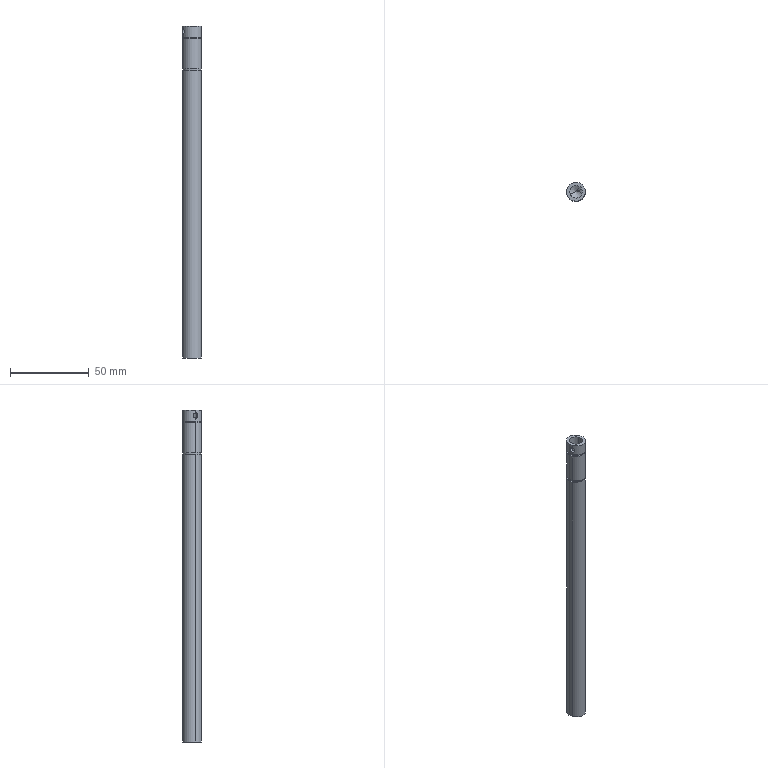Component | SolidWorks | TAR-02-025PaperFeedMotorAxis-1 | 1 solid | 26 faces | box 12 x 12 x 210.2 mm | volume 21464 mm3 | cylinder 16 | plane 6 | cone 4 | commonest cylinder face diameters 12 x6 11 x4 5 x2 3.3 x2 8 x2
build123d program:
from build123d import *

# Parameters (mm, degrees)
SKETCH1_R                     = 6
BOSS_EXTRUDE1_DEPTH           = 7
SKETCH2_R                     = 5.5
BOSS_EXTRUDE2_DEPTH           = 1.1
SKETCH3_R                     = 6
BOSS_EXTRUDE3_DEPTH           = 19
SKETCH4_R                     = 5.5
BOSS_EXTRUDE4_DEPTH           = 1.1
SKETCH5_R                     = 6
BOSS_EXTRUDE5_DEPTH           = 182
SIZE_MM_DOWEL_PIN_HOLE1_D     = 8
SIZE_MM_DOWEL_PIN_HOLE1_DEPTH = 36
SIZE_MM_DOWEL_PIN_HOLE1_TIP   = 2.403
M4_TAPPED_HOLE1_D             = 3.3
M4_TAPPED_HOLE1_DEPTH         = 5
M4_TAPPED_HOLE1_TIP           = 0.9914
M6_TAPPED_HOLE1_D             = 5
M6_TAPPED_HOLE1_DEPTH         = 20
M6_TAPPED_HOLE1_TIP           = 1.502


with BuildPart() as part:
    # Sketch1 → Boss-Extrude1 (new body)
    with BuildSketch(Plane.XY):
        Circle(SKETCH1_R)
    extrude(amount=BOSS_EXTRUDE1_DEPTH)

    # Sketch2 → Boss-Extrude2 (add)
    with BuildSketch(Plane.XY.offset(7)):
        Circle(SKETCH2_R)
    extrude(amount=BOSS_EXTRUDE2_DEPTH)

    # Sketch3 → Boss-Extrude3 (add)
    with BuildSketch(Plane.XY.offset(8.1)):
        Circle(SKETCH3_R)
    extrude(amount=BOSS_EXTRUDE3_DEPTH)

    # Sketch4 → Boss-Extrude4 (add)
    with BuildSketch(Plane.XY.offset(27.1)):
        Circle(SKETCH4_R)
    extrude(amount=BOSS_EXTRUDE4_DEPTH)

    # Sketch5 → Boss-Extrude5 (add)
    with BuildSketch(Plane.XY.offset(28.2)):
        Circle(SKETCH5_R)
    extrude(amount=BOSS_EXTRUDE5_DEPTH)

    # Size mm Dowel Pin Hole1
    with Locations(Plane(origin=(0, 0, 0), x_dir=(-1, 0, 0), z_dir=(0, 0, -1))):
        with Locations((0, 0)):
            Hole(SIZE_MM_DOWEL_PIN_HOLE1_D / 2, depth=SIZE_MM_DOWEL_PIN_HOLE1_DEPTH)
            with Locations((0, 0, -(SIZE_MM_DOWEL_PIN_HOLE1_DEPTH + SIZE_MM_DOWEL_PIN_HOLE1_TIP / 2))):  # 118° drill point
                Cone(0, SIZE_MM_DOWEL_PIN_HOLE1_D / 2, SIZE_MM_DOWEL_PIN_HOLE1_TIP, mode=Mode.SUBTRACT)

    # M4 Tapped Hole1
    with Locations(Plane(origin=(-6, 0, 3.5), x_dir=(0, 0, -1), z_dir=(-1, 0, 0))):
        with Locations((0, 0)):
            Hole(M4_TAPPED_HOLE1_D / 2, depth=M4_TAPPED_HOLE1_DEPTH)
            with Locations((0, 0, -(M4_TAPPED_HOLE1_DEPTH + M4_TAPPED_HOLE1_TIP / 2))):  # 118° drill point
                Cone(0, M4_TAPPED_HOLE1_D / 2, M4_TAPPED_HOLE1_TIP, mode=Mode.SUBTRACT)

    # M6 Tapped Hole1
    with Locations(Plane.XY.offset(210.2)):
        with Locations((0, 0)):
            Hole(M6_TAPPED_HOLE1_D / 2, depth=M6_TAPPED_HOLE1_DEPTH)
            with Locations((0, 0, -(M6_TAPPED_HOLE1_DEPTH + M6_TAPPED_HOLE1_TIP / 2))):  # 118° drill point
                Cone(0, M6_TAPPED_HOLE1_D / 2, M6_TAPPED_HOLE1_TIP, mode=Mode.SUBTRACT)


solid = part.part

# Placed as in the assembly
solid = solid.moved(Location((14.609, 9.288, 17.6), (-180, 0, -22.523)))
STEP:
#1=COLOUR_RGB('',0.7922,0.8196,0.9333);
#2=FILL_AREA_STYLE_COLOUR('',#1);
#3=FILL_AREA_STYLE('',(#2));
#4=SURFACE_STYLE_FILL_AREA(#3);
#5=SURFACE_SIDE_STYLE('',(#4));
#6=SURFACE_STYLE_USAGE(.BOTH.,#5);
#7=PRESENTATION_STYLE_ASSIGNMENT((#6));
#8=CARTESIAN_POINT('',(0.4842,0.328,-6.795));
#9=VERTEX_POINT('',#8);
#10=CARTESIAN_POINT('',(0.6661,0.4034,-6.795));
#11=VERTEX_POINT('',#10);
#12=CARTESIAN_POINT('',(0.5752,0.3657,-6.795));
#13=DIRECTION('',(0.,0.,-1.));
#14=DIRECTION('',(0.9237,0.383,0.));
#15=AXIS2_PLACEMENT_3D('',#12,#13,#14);
#16=CIRCLE('',#15,0.09843);
#17=EDGE_CURVE('',#9,#11,#16,.T.);
#18=ORIENTED_EDGE('',*,*,#17,.F.);
#19=CARTESIAN_POINT('',(0.4842,0.328,-7.583));
#20=VERTEX_POINT('',#19);
#21=CARTESIAN_POINT('',(0.4842,0.328,-7.583));
#22=DIRECTION('',(0.,0.,-1.));
#23=VECTOR('',#22,39.37);
#24=LINE('',#21,#23);
#25=EDGE_CURVE('',#9,#20,#24,.T.);
#26=ORIENTED_EDGE('',*,*,#25,.T.);
#27=CARTESIAN_POINT('',(0.6661,0.4034,-7.583));
#28=VERTEX_POINT('',#27);
#29=CARTESIAN_POINT('',(0.5752,0.3657,-7.583));
#30=DIRECTION('',(0.,0.,-1.));
#31=DIRECTION('',(0.9237,0.383,0.));
#32=AXIS2_PLACEMENT_3D('',#29,#30,#31);
#33=CIRCLE('',#32,0.09843);
#34=EDGE_CURVE('',#20,#28,#33,.T.);
#35=ORIENTED_EDGE('',*,*,#34,.T.);
#36=CARTESIAN_POINT('',(0.6661,0.4034,-7.583));
#37=DIRECTION('',(0.,0.,-1.));
#38=VECTOR('',#37,39.37);
#39=LINE('',#36,#38);
#40=EDGE_CURVE('',#11,#28,#39,.T.);
#41=ORIENTED_EDGE('',*,*,#40,.F.);
#42=EDGE_LOOP('',(#18,#26,#35,#41));
#43=FACE_OUTER_BOUND('',#42,.T.);
#44=CARTESIAN_POINT('',(0.5752,0.3657,-7.583));
#45=DIRECTION('',(0.,0.,-1.));
#46=DIRECTION('',(0.9237,0.383,0.));
#47=AXIS2_PLACEMENT_3D('',#44,#45,#46);
#48=CYLINDRICAL_SURFACE('',#47,0.09843);
#49=ADVANCED_FACE('',(#43),#48,.F.);
#50=CARTESIAN_POINT('',(0.5752,0.3657,-6.736));
#51=VERTEX_POINT('',#50);
#52=CARTESIAN_POINT('',(0.6661,0.4034,-6.795));
#53=DIRECTION('',(0.7918,0.3283,-0.515));
#54=VECTOR('',#53,39.37);
#55=LINE('',#52,#54);
#56=EDGE_CURVE('',#51,#11,#55,.T.);
#57=ORIENTED_EDGE('',*,*,#56,.F.);
#58=CARTESIAN_POINT('',(0.4842,0.328,-6.795));
#59=DIRECTION('',(-0.7918,-0.3283,-0.515));
#60=VECTOR('',#59,39.37);
#61=LINE('',#58,#60);
#62=EDGE_CURVE('',#51,#9,#61,.T.);
#63=ORIENTED_EDGE('',*,*,#62,.T.);
#64=ORIENTED_EDGE('',*,*,#17,.T.);
#65=EDGE_LOOP('',(#57,#63,#64));
#66=FACE_OUTER_BOUND('',#65,.T.);
#67=CARTESIAN_POINT('',(0.5752,0.3657,-6.795));
#68=DIRECTION('',(0.,0.,-1.));
#69=DIRECTION('',(0.9237,0.383,0.));
#70=AXIS2_PLACEMENT_3D('',#67,#68,#69);
#71=CONICAL_SURFACE('',#70,0.09843,1.03);
#72=ADVANCED_FACE('',(#66),#71,.F.);
#73=CARTESIAN_POINT('',(0.4297,0.3053,0.6201));
#74=VERTEX_POINT('',#73);
#75=CARTESIAN_POINT('',(0.4297,0.3053,0.4902));
#76=VERTEX_POINT('',#75);
#77=CARTESIAN_POINT('',(0.4297,0.3053,0.6201));
#78=CARTESIAN_POINT('',(0.4281,0.3093,0.6201));
#79=CARTESIAN_POINT('',(0.4266,0.3134,0.6196));
#80=CARTESIAN_POINT('',(0.424,0.3214,0.618));
#81=CARTESIAN_POINT('',(0.4229,0.3253,0.6167));
#82=CARTESIAN_POINT('',(0.4201,0.337,0.6118));
#83=CARTESIAN_POINT('',(0.419,0.3442,0.607));
#84=CARTESIAN_POINT('',(0.4181,0.3535,0.598));
#85=CARTESIAN_POINT('',(0.4179,0.3563,0.5948));
#86=CARTESIAN_POINT('',(0.4177,0.3613,0.5878));
#87=CARTESIAN_POINT('',(0.4177,0.3635,0.584));
#88=CARTESIAN_POINT('',(0.4177,0.367,0.5762));
#89=CARTESIAN_POINT('',(0.4177,0.3684,0.5721));
#90=CARTESIAN_POINT('',(0.4177,0.3702,0.5638));
#91=CARTESIAN_POINT('',(0.4178,0.3707,0.5594));
#92=CARTESIAN_POINT('',(0.4178,0.3707,0.5466));
#93=CARTESIAN_POINT('',(0.4177,0.3688,0.5379));
#94=CARTESIAN_POINT('',(0.4177,0.3635,0.5262));
#95=CARTESIAN_POINT('',(0.4177,0.3613,0.5224));
#96=CARTESIAN_POINT('',(0.4179,0.3563,0.5154));
#97=CARTESIAN_POINT('',(0.4181,0.3535,0.5122));
#98=CARTESIAN_POINT('',(0.4187,0.3473,0.5062));
#99=CARTESIAN_POINT('',(0.4191,0.3439,0.5035));
#100=CARTESIAN_POINT('',(0.4203,0.3369,0.4988));
#101=CARTESIAN_POINT('',(0.421,0.3331,0.4968));
#102=CARTESIAN_POINT('',(0.4238,0.3214,0.4919));
#103=CARTESIAN_POINT('',(0.4264,0.3134,0.4902));
#104=CARTESIAN_POINT('',(0.4297,0.3053,0.4902));
#105=B_SPLINE_CURVE_WITH_KNOTS('',3,(#77,#78,#79,#80,#81,#82,#83,#84,#85,#86,#87,#88,#89,#90,#91,#92,#93,#94,#95,#96,#97,#98,#99,#100,#101,#102,#103,#104),.UNSPECIFIED.,.F.,.F.,(4,2,2,2,2,2,2,2,2,2,2,2,2,4),(0.005218,0.005543,0.005869,0.006521,0.006847,0.007173,0.007499,0.007824,0.008476,0.008802,0.009128,0.009454,0.009779,0.01043),.UNSPECIFIED.);
#106=EDGE_CURVE('',#74,#76,#105,.T.);
#107=ORIENTED_EDGE('',*,*,#106,.F.);
#108=CARTESIAN_POINT('',(0.357,0.2752,0.6201));
#109=VERTEX_POINT('',#108);
#110=CARTESIAN_POINT('',(0.357,0.2752,0.6201));
#111=DIRECTION('',(-0.9237,-0.383,0.));
#112=VECTOR('',#111,39.37);
#113=LINE('',#110,#112);
#114=EDGE_CURVE('',#74,#109,#113,.T.);
#115=ORIENTED_EDGE('',*,*,#114,.T.);
#116=CARTESIAN_POINT('',(0.357,0.2752,0.4902));
#117=VERTEX_POINT('',#116);
#118=CARTESIAN_POINT('',(0.357,0.2752,0.4902));
#119=CARTESIAN_POINT('',(0.3553,0.2792,0.4902));
#120=CARTESIAN_POINT('',(0.3538,0.2831,0.4906));
#121=CARTESIAN_POINT('',(0.351,0.291,0.4922));
#122=CARTESIAN_POINT('',(0.3497,0.2949,0.4935));
#123=CARTESIAN_POINT('',(0.3475,0.3025,0.4968));
#124=CARTESIAN_POINT('',(0.3465,0.3061,0.4988));
#125=CARTESIAN_POINT('',(0.3448,0.3131,0.5035));
#126=CARTESIAN_POINT('',(0.3441,0.3164,0.5062));
#127=CARTESIAN_POINT('',(0.3423,0.3253,0.5152));
#128=CARTESIAN_POINT('',(0.3416,0.3302,0.5224));
#129=CARTESIAN_POINT('',(0.3407,0.3369,0.538));
#130=CARTESIAN_POINT('',(0.3405,0.3387,0.5466));
#131=CARTESIAN_POINT('',(0.3405,0.3387,0.5593));
#132=CARTESIAN_POINT('',(0.3405,0.3382,0.5637));
#133=CARTESIAN_POINT('',(0.3407,0.3365,0.572));
#134=CARTESIAN_POINT('',(0.3409,0.3352,0.5761));
#135=CARTESIAN_POINT('',(0.3416,0.3302,0.5879));
#136=CARTESIAN_POINT('',(0.3423,0.3253,0.5951));
#137=CARTESIAN_POINT('',(0.3441,0.3163,0.6041));
#138=CARTESIAN_POINT('',(0.3448,0.3131,0.6067));
#139=CARTESIAN_POINT('',(0.3465,0.3062,0.6114));
#140=CARTESIAN_POINT('',(0.3475,0.3025,0.6135));
#141=CARTESIAN_POINT('',(0.3497,0.2949,0.6167));
#142=CARTESIAN_POINT('',(0.351,0.291,0.618));
#143=CARTESIAN_POINT('',(0.3538,0.2831,0.6197));
#144=CARTESIAN_POINT('',(0.3553,0.2791,0.6201));
#145=CARTESIAN_POINT('',(0.357,0.2752,0.6201));
#146=B_SPLINE_CURVE_WITH_KNOTS('',3,(#118,#119,#120,#121,#122,#123,#124,#125,#126,#127,#128,#129,#130,#131,#132,#133,#134,#135,#136,#137,#138,#139,#140,#141,#142,#143,#144,#145),.UNSPECIFIED.,.F.,.F.,(4,2,2,2,2,2,2,2,2,2,2,2,2,4),(0.,0.000324,0.000648,0.000972,0.001296,0.001944,0.002592,0.002916,0.00324,0.003888,0.004212,0.004536,0.00486,0.005184),.UNSPECIFIED.);
#147=EDGE_CURVE('',#117,#109,#146,.T.);
#148=ORIENTED_EDGE('',*,*,#147,.F.);
#149=CARTESIAN_POINT('',(0.357,0.2752,0.4902));
#150=DIRECTION('',(-0.9237,-0.383,0.));
#151=VECTOR('',#150,39.37);
#152=LINE('',#149,#151);
#153=EDGE_CURVE('',#76,#117,#152,.T.);
#154=ORIENTED_EDGE('',*,*,#153,.F.);
#155=EDGE_LOOP('',(#107,#115,#148,#154));
#156=FACE_OUTER_BOUND('',#155,.T.);
#157=CARTESIAN_POINT('',(0.357,0.2752,0.5551));
#158=DIRECTION('',(-0.9237,-0.383,0.));
#159=DIRECTION('',(0.,0.,-1.));
#160=AXIS2_PLACEMENT_3D('',#157,#158,#159);
#161=CYLINDRICAL_SURFACE('',#160,0.06496);
#162=ADVANCED_FACE('',(#156),#161,.F.);
#163=CARTESIAN_POINT('',(0.7206,0.426,-0.7244));
#164=VERTEX_POINT('',#163);
#165=CARTESIAN_POINT('',(0.4297,0.3053,-0.7244));
#166=VERTEX_POINT('',#165);
#167=CARTESIAN_POINT('',(0.5752,0.3657,-0.7244));
#168=DIRECTION('',(0.,0.,1.));
#169=DIRECTION('',(-0.9237,-0.383,0.));
#170=AXIS2_PLACEMENT_3D('',#167,#168,#169);
#171=CIRCLE('',#170,0.1575);
#172=EDGE_CURVE('',#164,#166,#171,.T.);
#173=ORIENTED_EDGE('',*,*,#172,.F.);
#174=CARTESIAN_POINT('',(0.7206,0.426,0.6929));
#175=VERTEX_POINT('',#174);
#176=CARTESIAN_POINT('',(0.7206,0.426,0.6929));
#177=DIRECTION('',(0.,0.,1.));
#178=VECTOR('',#177,39.37);
#179=LINE('',#176,#178);
#180=EDGE_CURVE('',#164,#175,#179,.T.);
#181=ORIENTED_EDGE('',*,*,#180,.T.);
#182=CARTESIAN_POINT('',(0.4297,0.3053,0.6929));
#183=VERTEX_POINT('',#182);
#184=CARTESIAN_POINT('',(0.5752,0.3657,0.6929));
#185=DIRECTION('',(0.,0.,1.));
#186=DIRECTION('',(-0.9237,-0.383,0.));
#187=AXIS2_PLACEMENT_3D('',#184,#185,#186);
#188=CIRCLE('',#187,0.1575);
#189=EDGE_CURVE('',#175,#183,#188,.T.);
#190=ORIENTED_EDGE('',*,*,#189,.T.);
#191=CARTESIAN_POINT('',(0.4297,0.3053,0.6929));
#192=DIRECTION('',(0.,0.,1.));
#193=VECTOR('',#192,39.37);
#194=LINE('',#191,#193);
#195=EDGE_CURVE('',#74,#183,#194,.T.);
#196=ORIENTED_EDGE('',*,*,#195,.F.);
#197=ORIENTED_EDGE('',*,*,#106,.T.);
#198=CARTESIAN_POINT('',(0.4297,0.3053,0.6929));
#199=DIRECTION('',(0.,0.,1.));
#200=VECTOR('',#199,39.37);
#201=LINE('',#198,#200);
#202=EDGE_CURVE('',#166,#76,#201,.T.);
#203=ORIENTED_EDGE('',*,*,#202,.F.);
#204=EDGE_LOOP('',(#173,#181,#190,#196,#197,#203));
#205=FACE_OUTER_BOUND('',#204,.T.);
#206=CARTESIAN_POINT('',(0.5752,0.3657,0.6929));
#207=DIRECTION('',(0.,0.,1.));
#208=DIRECTION('',(-0.9237,-0.383,0.));
#209=AXIS2_PLACEMENT_3D('',#206,#207,#208);
#210=CYLINDRICAL_SURFACE('',#209,0.1575);
#211=ADVANCED_FACE('',(#205),#210,.F.);
#212=CARTESIAN_POINT('',(0.5752,0.3657,-0.819));
#213=VERTEX_POINT('',#212);
#214=CARTESIAN_POINT('',(0.4297,0.3053,-0.7244));
#215=DIRECTION('',(-0.7918,-0.3283,0.515));
#216=VECTOR('',#215,39.37);
#217=LINE('',#214,#216);
#218=EDGE_CURVE('',#213,#166,#217,.T.);
#219=ORIENTED_EDGE('',*,*,#218,.F.);
#220=CARTESIAN_POINT('',(0.7206,0.426,-0.7244));
#221=DIRECTION('',(0.7918,0.3283,0.515));
#222=VECTOR('',#221,39.37);
#223=LINE('',#220,#222);
#224=EDGE_CURVE('',#213,#164,#223,.T.);
#225=ORIENTED_EDGE('',*,*,#224,.T.);
#226=ORIENTED_EDGE('',*,*,#172,.T.);
#227=EDGE_LOOP('',(#219,#225,#226));
#228=FACE_OUTER_BOUND('',#227,.T.);
#229=CARTESIAN_POINT('',(0.5752,0.3657,-0.7244));
#230=DIRECTION('',(0.,0.,1.));
#231=DIRECTION('',(-0.9237,-0.383,0.));
#232=AXIS2_PLACEMENT_3D('',#229,#230,#231);
#233=CONICAL_SURFACE('',#232,0.1575,1.03);
#234=ADVANCED_FACE('',(#228),#233,.F.);
#235=CARTESIAN_POINT('',(0.7934,0.4561,-7.583));
#236=VERTEX_POINT('',#235);
#237=CARTESIAN_POINT('',(0.357,0.2752,-7.583));
#238=VERTEX_POINT('',#237);
#239=CARTESIAN_POINT('',(0.5752,0.3657,-7.583));
#240=DIRECTION('',(0.,0.,-1.));
#241=DIRECTION('',(0.9237,0.383,0.));
#242=AXIS2_PLACEMENT_3D('',#239,#240,#241);
#243=CIRCLE('',#242,0.2362);
#244=EDGE_CURVE('',#236,#238,#243,.T.);
#245=ORIENTED_EDGE('',*,*,#244,.F.);
#246=CARTESIAN_POINT('',(0.7934,0.4561,-0.4173));
#247=VERTEX_POINT('',#246);
#248=CARTESIAN_POINT('',(0.7934,0.4561,-7.583));
#249=DIRECTION('',(0.,0.,1.));
#250=VECTOR('',#249,39.37);
#251=LINE('',#248,#250);
#252=EDGE_CURVE('',#236,#247,#251,.T.);
#253=ORIENTED_EDGE('',*,*,#252,.T.);
#254=CARTESIAN_POINT('',(0.357,0.2752,-0.4173));
#255=VERTEX_POINT('',#254);
#256=CARTESIAN_POINT('',(0.5752,0.3657,-0.4173));
#257=DIRECTION('',(0.,0.,-1.));
#258=DIRECTION('',(0.9237,0.383,0.));
#259=AXIS2_PLACEMENT_3D('',#256,#257,#258);
#260=CIRCLE('',#259,0.2362);
#261=EDGE_CURVE('',#247,#255,#260,.T.);
#262=ORIENTED_EDGE('',*,*,#261,.T.);
#263=CARTESIAN_POINT('',(0.357,0.2752,-7.583));
#264=DIRECTION('',(0.,0.,1.));
#265=VECTOR('',#264,39.37);
#266=LINE('',#263,#265);
#267=EDGE_CURVE('',#238,#255,#266,.T.);
#268=ORIENTED_EDGE('',*,*,#267,.F.);
#269=EDGE_LOOP('',(#245,#253,#262,#268));
#270=FACE_OUTER_BOUND('',#269,.T.);
#271=CARTESIAN_POINT('',(0.5752,0.3657,-7.583));
#272=DIRECTION('',(0.,0.,1.));
#273=DIRECTION('',(-0.9237,-0.383,0.));
#274=AXIS2_PLACEMENT_3D('',#271,#272,#273);
#275=CYLINDRICAL_SURFACE('',#274,0.2362);
#276=ADVANCED_FACE('',(#270),#275,.T.);
#277=CARTESIAN_POINT('',(0.7752,0.4486,-0.4173));
#278=VERTEX_POINT('',#277);
#279=CARTESIAN_POINT('',(0.3751,0.2827,-0.4173));
#280=VERTEX_POINT('',#279);
#281=CARTESIAN_POINT('',(0.5752,0.3657,-0.4173));
#282=DIRECTION('',(0.,0.,-1.));
#283=DIRECTION('',(0.9237,0.383,0.));
#284=AXIS2_PLACEMENT_3D('',#281,#282,#283);
#285=CIRCLE('',#284,0.2165);
#286=EDGE_CURVE('',#278,#280,#285,.T.);
#287=ORIENTED_EDGE('',*,*,#286,.F.);
#288=CARTESIAN_POINT('',(0.7752,0.4486,-0.374));
#289=VERTEX_POINT('',#288);
#290=CARTESIAN_POINT('',(0.7752,0.4486,-0.4173));
#291=DIRECTION('',(0.,0.,1.));
#292=VECTOR('',#291,39.37);
#293=LINE('',#290,#292);
#294=EDGE_CURVE('',#278,#289,#293,.T.);
#295=ORIENTED_EDGE('',*,*,#294,.T.);
#296=CARTESIAN_POINT('',(0.3751,0.2827,-0.374));
#297=VERTEX_POINT('',#296);
#298=CARTESIAN_POINT('',(0.5752,0.3657,-0.374));
#299=DIRECTION('',(0.,0.,-1.));
#300=DIRECTION('',(0.9237,0.383,0.));
#301=AXIS2_PLACEMENT_3D('',#298,#299,#300);
#302=CIRCLE('',#301,0.2165);
#303=EDGE_CURVE('',#289,#297,#302,.T.);
#304=ORIENTED_EDGE('',*,*,#303,.T.);
#305=CARTESIAN_POINT('',(0.3751,0.2827,-0.4173));
#306=DIRECTION('',(0.,0.,1.));
#307=VECTOR('',#306,39.37);
#308=LINE('',#305,#307);
#309=EDGE_CURVE('',#280,#297,#308,.T.);
#310=ORIENTED_EDGE('',*,*,#309,.F.);
#311=EDGE_LOOP('',(#287,#295,#304,#310));
#312=FACE_OUTER_BOUND('',#311,.T.);
#313=CARTESIAN_POINT('',(0.5752,0.3657,-0.4173));
#314=DIRECTION('',(0.,0.,1.));
#315=DIRECTION('',(-0.9237,-0.383,0.));
#316=AXIS2_PLACEMENT_3D('',#313,#314,#315);
#317=CYLINDRICAL_SURFACE('',#316,0.2165);
#318=ADVANCED_FACE('',(#312),#317,.T.);
#319=CARTESIAN_POINT('',(0.7934,0.4561,-0.374));
#320=VERTEX_POINT('',#319);
#321=CARTESIAN_POINT('',(0.357,0.2752,-0.374));
#322=VERTEX_POINT('',#321);
#323=CARTESIAN_POINT('',(0.5752,0.3657,-0.374));
#324=DIRECTION('',(0.,0.,-1.));
#325=DIRECTION('',(0.9237,0.383,0.));
#326=AXIS2_PLACEMENT_3D('',#323,#324,#325);
#327=CIRCLE('',#326,0.2362);
#328=EDGE_CURVE('',#320,#322,#327,.T.);
#329=ORIENTED_EDGE('',*,*,#328,.F.);
#330=CARTESIAN_POINT('',(0.7934,0.4561,0.374));
#331=VERTEX_POINT('',#330);
#332=CARTESIAN_POINT('',(0.7934,0.4561,-0.374));
#333=DIRECTION('',(0.,0.,1.));
#334=VECTOR('',#333,39.37);
#335=LINE('',#332,#334);
#336=EDGE_CURVE('',#320,#331,#335,.T.);
#337=ORIENTED_EDGE('',*,*,#336,.T.);
#338=CARTESIAN_POINT('',(0.357,0.2752,0.374));
#339=VERTEX_POINT('',#338);
#340=CARTESIAN_POINT('',(0.5752,0.3657,0.374));
#341=DIRECTION('',(0.,0.,-1.));
#342=DIRECTION('',(0.9237,0.383,0.));
#343=AXIS2_PLACEMENT_3D('',#340,#341,#342);
#344=CIRCLE('',#343,0.2362);
#345=EDGE_CURVE('',#331,#339,#344,.T.);
#346=ORIENTED_EDGE('',*,*,#345,.T.);
#347=CARTESIAN_POINT('',(0.357,0.2752,-0.374));
#348=DIRECTION('',(0.,0.,1.));
#349=VECTOR('',#348,39.37);
#350=LINE('',#347,#349);
#351=EDGE_CURVE('',#322,#339,#350,.T.);
#352=ORIENTED_EDGE('',*,*,#351,.F.);
#353=EDGE_LOOP('',(#329,#337,#346,#352));
#354=FACE_OUTER_BOUND('',#353,.T.);
#355=CARTESIAN_POINT('',(0.5752,0.3657,-0.374));
#356=DIRECTION('',(0.,0.,1.));
#357=DIRECTION('',(-0.9237,-0.383,0.));
#358=AXIS2_PLACEMENT_3D('',#355,#356,#357);
#359=CYLINDRICAL_SURFACE('',#358,0.2362);
#360=ADVANCED_FACE('',(#354),#359,.T.);
#361=CARTESIAN_POINT('',(0.7752,0.4486,0.374));
#362=VERTEX_POINT('',#361);
#363=CARTESIAN_POINT('',(0.3751,0.2827,0.374));
#364=VERTEX_POINT('',#363);
#365=CARTESIAN_POINT('',(0.5752,0.3657,0.374));
#366=DIRECTION('',(0.,0.,-1.));
#367=DIRECTION('',(0.9237,0.383,0.));
#368=AXIS2_PLACEMENT_3D('',#365,#366,#367);
#369=CIRCLE('',#368,0.2165);
#370=EDGE_CURVE('',#362,#364,#369,.T.);
#371=ORIENTED_EDGE('',*,*,#370,.F.);
#372=CARTESIAN_POINT('',(0.7752,0.4486,0.4173));
#373=VERTEX_POINT('',#372);
#374=CARTESIAN_POINT('',(0.7752,0.4486,0.374));
#375=DIRECTION('',(0.,0.,1.));
#376=VECTOR('',#375,39.37);
#377=LINE('',#374,#376);
#378=EDGE_CURVE('',#362,#373,#377,.T.);
#379=ORIENTED_EDGE('',*,*,#378,.T.);
#380=CARTESIAN_POINT('',(0.3751,0.2827,0.4173));
#381=VERTEX_POINT('',#380);
#382=CARTESIAN_POINT('',(0.5752,0.3657,0.4173));
#383=DIRECTION('',(0.,0.,-1.));
#384=DIRECTION('',(0.9237,0.383,0.));
#385=AXIS2_PLACEMENT_3D('',#382,#383,#384);
#386=CIRCLE('',#385,0.2165);
#387=EDGE_CURVE('',#373,#381,#386,.T.);
#388=ORIENTED_EDGE('',*,*,#387,.T.);
#389=CARTESIAN_POINT('',(0.3751,0.2827,0.374));
#390=DIRECTION('',(0.,0.,1.));
#391=VECTOR('',#390,39.37);
#392=LINE('',#389,#391);
#393=EDGE_CURVE('',#364,#381,#392,.T.);
#394=ORIENTED_EDGE('',*,*,#393,.F.);
#395=EDGE_LOOP('',(#371,#379,#388,#394));
#396=FACE_OUTER_BOUND('',#395,.T.);
#397=CARTESIAN_POINT('',(0.5752,0.3657,0.374));
#398=DIRECTION('',(0.,0.,1.));
#399=DIRECTION('',(-0.9237,-0.383,0.));
#400=AXIS2_PLACEMENT_3D('',#397,#398,#399);
#401=CYLINDRICAL_SURFACE('',#400,0.2165);
#402=ADVANCED_FACE('',(#396),#401,.T.);
#403=CARTESIAN_POINT('',(0.7934,0.4561,0.4173));
#404=VERTEX_POINT('',#403);
#405=CARTESIAN_POINT('',(0.357,0.2752,0.4173));
#406=VERTEX_POINT('',#405);
#407=CARTESIAN_POINT('',(0.5752,0.3657,0.4173));
#408=DIRECTION('',(0.,0.,-1.));
#409=DIRECTION('',(0.9237,0.383,0.));
#410=AXIS2_PLACEMENT_3D('',#407,#408,#409);
#411=CIRCLE('',#410,0.2362);
#412=EDGE_CURVE('',#404,#406,#411,.T.);
#413=ORIENTED_EDGE('',*,*,#412,.F.);
#414=CARTESIAN_POINT('',(0.7934,0.4561,0.6929));
#415=VERTEX_POINT('',#414);
#416=CARTESIAN_POINT('',(0.7934,0.4561,0.4173));
#417=DIRECTION('',(0.,0.,1.));
#418=VECTOR('',#417,39.37);
#419=LINE('',#416,#418);
#420=EDGE_CURVE('',#404,#415,#419,.T.);
#421=ORIENTED_EDGE('',*,*,#420,.T.);
#422=CARTESIAN_POINT('',(0.357,0.2752,0.6929));
#423=VERTEX_POINT('',#422);
#424=CARTESIAN_POINT('',(0.5752,0.3657,0.6929));
#425=DIRECTION('',(0.,0.,-1.));
#426=DIRECTION('',(0.9237,0.383,0.));
#427=AXIS2_PLACEMENT_3D('',#424,#425,#426);
#428=CIRCLE('',#427,0.2362);
#429=EDGE_CURVE('',#415,#423,#428,.T.);
#430=ORIENTED_EDGE('',*,*,#429,.T.);
#431=CARTESIAN_POINT('',(0.357,0.2752,0.4173));
#432=DIRECTION('',(0.,0.,1.));
#433=VECTOR('',#432,39.37);
#434=LINE('',#431,#433);
#435=EDGE_CURVE('',#109,#423,#434,.T.);
#436=ORIENTED_EDGE('',*,*,#435,.F.);
#437=CARTESIAN_POINT('',(0.357,0.2752,0.6201));
#438=CARTESIAN_POINT('',(0.3602,0.2673,0.6201));
#439=CARTESIAN_POINT('',(0.364,0.2596,0.6184));
#440=CARTESIAN_POINT('',(0.3696,0.2492,0.6135));
#441=CARTESIAN_POINT('',(0.3715,0.2459,0.6114));
#442=CARTESIAN_POINT('',(0.3752,0.2398,0.6067));
#443=CARTESIAN_POINT('',(0.377,0.237,0.6041));
#444=CARTESIAN_POINT('',(0.3804,0.2319,0.5981));
#445=CARTESIAN_POINT('',(0.382,0.2297,0.5948));
#446=CARTESIAN_POINT('',(0.3848,0.2257,0.5877));
#447=CARTESIAN_POINT('',(0.3861,0.2241,0.584));
#448=CARTESIAN_POINT('',(0.3881,0.2214,0.5761));
#449=CARTESIAN_POINT('',(0.3889,0.2204,0.572));
#450=CARTESIAN_POINT('',(0.39,0.219,0.5637));
#451=CARTESIAN_POINT('',(0.3903,0.2187,0.5594));
#452=CARTESIAN_POINT('',(0.3903,0.2187,0.5508));
#453=CARTESIAN_POINT('',(0.39,0.219,0.5466));
#454=CARTESIAN_POINT('',(0.3889,0.2204,0.5383));
#455=CARTESIAN_POINT('',(0.3881,0.2214,0.5341));
#456=CARTESIAN_POINT('',(0.3851,0.2254,0.5224));
#457=CARTESIAN_POINT('',(0.3821,0.2294,0.5152));
#458=CARTESIAN_POINT('',(0.3754,0.2395,0.5032));
#459=CARTESIAN_POINT('',(0.3715,0.2457,0.4984));
#460=CARTESIAN_POINT('',(0.3659,0.2561,0.4935));
#461=CARTESIAN_POINT('',(0.364,0.2598,0.4923));
#462=CARTESIAN_POINT('',(0.3603,0.2673,0.4906));
#463=CARTESIAN_POINT('',(0.3586,0.2712,0.4902));
#464=CARTESIAN_POINT('',(0.357,0.2752,0.4902));
#465=B_SPLINE_CURVE_WITH_KNOTS('',3,(#437,#438,#439,#440,#441,#442,#443,#444,#445,#446,#447,#448,#449,#450,#451,#452,#453,#454,#455,#456,#457,#458,#459,#460,#461,#462,#463,#464),.UNSPECIFIED.,.F.,.F.,(4,2,2,2,2,2,2,2,2,2,2,2,2,4),(0.005184,0.005832,0.006155,0.006479,0.006803,0.007127,0.007451,0.007775,0.008099,0.008423,0.00907,0.009718,0.01004,0.01037),.UNSPECIFIED.);
#466=EDGE_CURVE('',#109,#117,#465,.T.);
#467=ORIENTED_EDGE('',*,*,#466,.T.);
#468=CARTESIAN_POINT('',(0.357,0.2752,0.4173));
#469=DIRECTION('',(0.,0.,1.));
#470=VECTOR('',#469,39.37);
#471=LINE('',#468,#470);
#472=EDGE_CURVE('',#406,#117,#471,.T.);
#473=ORIENTED_EDGE('',*,*,#472,.F.);
#474=EDGE_LOOP('',(#413,#421,#430,#436,#467,#473));
#475=FACE_OUTER_BOUND('',#474,.T.);
#476=CARTESIAN_POINT('',(0.5752,0.3657,0.4173));
#477=DIRECTION('',(0.,0.,1.));
#478=DIRECTION('',(-0.9237,-0.383,0.));
#479=AXIS2_PLACEMENT_3D('',#476,#477,#478);
#480=CYLINDRICAL_SURFACE('',#479,0.2362);
#481=ADVANCED_FACE('',(#475),#480,.T.);
#482=ORIENTED_EDGE('',*,*,#420,.F.);
#483=CARTESIAN_POINT('',(0.5752,0.3657,0.4173));
#484=DIRECTION('',(0.,0.,-1.));
#485=DIRECTION('',(0.9237,0.383,0.));
#486=AXIS2_PLACEMENT_3D('',#483,#484,#485);
#487=CIRCLE('',#486,0.2362);
#488=EDGE_CURVE('',#406,#404,#487,.T.);
#489=ORIENTED_EDGE('',*,*,#488,.F.);
#490=ORIENTED_EDGE('',*,*,#472,.T.);
#491=ORIENTED_EDGE('',*,*,#147,.T.);
#492=ORIENTED_EDGE('',*,*,#435,.T.);
#493=CARTESIAN_POINT('',(0.5752,0.3657,0.6929));
#494=DIRECTION('',(0.,0.,-1.));
#495=DIRECTION('',(0.9237,0.383,0.));
#496=AXIS2_PLACEMENT_3D('',#493,#494,#495);
#497=CIRCLE('',#496,0.2362);
#498=EDGE_CURVE('',#423,#415,#497,.T.);
#499=ORIENTED_EDGE('',*,*,#498,.T.);
#500=EDGE_LOOP('',(#482,#489,#490,#491,#492,#499));
#501=FACE_OUTER_BOUND('',#500,.T.);
#502=CARTESIAN_POINT('',(0.5752,0.3657,0.4173));
#503=DIRECTION('',(0.,0.,1.));
#504=DIRECTION('',(-0.9237,-0.383,0.));
#505=AXIS2_PLACEMENT_3D('',#502,#503,#504);
#506=CYLINDRICAL_SURFACE('',#505,0.2362);
#507=ADVANCED_FACE('',(#501),#506,.T.);
#508=CARTESIAN_POINT('',(0.5752,0.3657,0.4173));
#509=DIRECTION('',(0.,0.,-1.));
#510=DIRECTION('',(0.9237,0.383,0.));
#511=AXIS2_PLACEMENT_3D('',#508,#509,#510);
#512=CIRCLE('',#511,0.2165);
#513=EDGE_CURVE('',#381,#373,#512,.T.);
#514=ORIENTED_EDGE('',*,*,#513,.F.);
#515=ORIENTED_EDGE('',*,*,#387,.F.);
#516=EDGE_LOOP('',(#514,#515));
#517=FACE_BOUND('',#516,.T.);
#518=ORIENTED_EDGE('',*,*,#488,.T.);
#519=ORIENTED_EDGE('',*,*,#412,.T.);
#520=EDGE_LOOP('',(#518,#519));
#521=FACE_OUTER_BOUND('',#520,.T.);
#522=CARTESIAN_POINT('',(0.5752,0.3657,0.4173));
#523=DIRECTION('',(0.,0.,-1.));
#524=DIRECTION('',(0.9237,0.383,0.));
#525=AXIS2_PLACEMENT_3D('',#522,#523,#524);
#526=PLANE('',#525);
#527=ADVANCED_FACE('',(#517,#521),#526,.T.);
#528=CARTESIAN_POINT('',(0.5752,0.3657,0.6929));
#529=DIRECTION('',(0.,0.,1.));
#530=DIRECTION('',(-0.9237,-0.383,0.));
#531=AXIS2_PLACEMENT_3D('',#528,#529,#530);
#532=CIRCLE('',#531,0.1575);
#533=EDGE_CURVE('',#183,#175,#532,.T.);
#534=ORIENTED_EDGE('',*,*,#533,.F.);
#535=ORIENTED_EDGE('',*,*,#189,.F.);
#536=EDGE_LOOP('',(#534,#535));
#537=FACE_BOUND('',#536,.T.);
#538=ORIENTED_EDGE('',*,*,#498,.F.);
#539=ORIENTED_EDGE('',*,*,#429,.F.);
#540=EDGE_LOOP('',(#538,#539));
#541=FACE_OUTER_BOUND('',#540,.T.);
#542=CARTESIAN_POINT('',(0.5752,0.3657,0.6929));
#543=DIRECTION('',(0.,0.,-1.));
#544=DIRECTION('',(0.9237,0.383,0.));
#545=AXIS2_PLACEMENT_3D('',#542,#543,#544);
#546=PLANE('',#545);
#547=ADVANCED_FACE('',(#537,#541),#546,.F.);
#548=ORIENTED_EDGE('',*,*,#378,.F.);
#549=CARTESIAN_POINT('',(0.5752,0.3657,0.374));
#550=DIRECTION('',(0.,0.,-1.));
#551=DIRECTION('',(0.9237,0.383,0.));
#552=AXIS2_PLACEMENT_3D('',#549,#550,#551);
#553=CIRCLE('',#552,0.2165);
#554=EDGE_CURVE('',#364,#362,#553,.T.);
#555=ORIENTED_EDGE('',*,*,#554,.F.);
#556=ORIENTED_EDGE('',*,*,#393,.T.);
#557=ORIENTED_EDGE('',*,*,#513,.T.);
#558=EDGE_LOOP('',(#548,#555,#556,#557));
#559=FACE_OUTER_BOUND('',#558,.T.);
#560=CARTESIAN_POINT('',(0.5752,0.3657,0.374));
#561=DIRECTION('',(0.,0.,1.));
#562=DIRECTION('',(-0.9237,-0.383,0.));
#563=AXIS2_PLACEMENT_3D('',#560,#561,#562);
#564=CYLINDRICAL_SURFACE('',#563,0.2165);
#565=ADVANCED_FACE('',(#559),#564,.T.);
#566=ORIENTED_EDGE('',*,*,#336,.F.);
#567=CARTESIAN_POINT('',(0.5752,0.3657,-0.374));
#568=DIRECTION('',(0.,0.,-1.));
#569=DIRECTION('',(0.9237,0.383,0.));
#570=AXIS2_PLACEMENT_3D('',#567,#568,#569);
#571=CIRCLE('',#570,0.2362);
#572=EDGE_CURVE('',#322,#320,#571,.T.);
#573=ORIENTED_EDGE('',*,*,#572,.F.);
#574=ORIENTED_EDGE('',*,*,#351,.T.);
#575=CARTESIAN_POINT('',(0.5752,0.3657,0.374));
#576=DIRECTION('',(0.,0.,-1.));
#577=DIRECTION('',(0.9237,0.383,0.));
#578=AXIS2_PLACEMENT_3D('',#575,#576,#577);
#579=CIRCLE('',#578,0.2362);
#580=EDGE_CURVE('',#339,#331,#579,.T.);
#581=ORIENTED_EDGE('',*,*,#580,.T.);
#582=EDGE_LOOP('',(#566,#573,#574,#581));
#583=FACE_OUTER_BOUND('',#582,.T.);
#584=CARTESIAN_POINT('',(0.5752,0.3657,-0.374));
#585=DIRECTION('',(0.,0.,1.));
#586=DIRECTION('',(-0.9237,-0.383,0.));
#587=AXIS2_PLACEMENT_3D('',#584,#585,#586);
#588=CYLINDRICAL_SURFACE('',#587,0.2362);
#589=ADVANCED_FACE('',(#583),#588,.T.);
#590=CARTESIAN_POINT('',(0.5752,0.3657,-0.374));
#591=DIRECTION('',(0.,0.,-1.));
#592=DIRECTION('',(0.9237,0.383,0.));
#593=AXIS2_PLACEMENT_3D('',#590,#591,#592);
#594=CIRCLE('',#593,0.2165);
#595=EDGE_CURVE('',#297,#289,#594,.T.);
#596=ORIENTED_EDGE('',*,*,#595,.F.);
#597=ORIENTED_EDGE('',*,*,#303,.F.);
#598=EDGE_LOOP('',(#596,#597));
#599=FACE_BOUND('',#598,.T.);
#600=ORIENTED_EDGE('',*,*,#572,.T.);
#601=ORIENTED_EDGE('',*,*,#328,.T.);
#602=EDGE_LOOP('',(#600,#601));
#603=FACE_OUTER_BOUND('',#602,.T.);
#604=CARTESIAN_POINT('',(0.5752,0.3657,-0.374));
#605=DIRECTION('',(0.,0.,-1.));
#606=DIRECTION('',(0.9237,0.383,0.));
#607=AXIS2_PLACEMENT_3D('',#604,#605,#606);
#608=PLANE('',#607);
#609=ADVANCED_FACE('',(#599,#603),#608,.T.);
#610=ORIENTED_EDGE('',*,*,#554,.T.);
#611=ORIENTED_EDGE('',*,*,#370,.T.);
#612=EDGE_LOOP('',(#610,#611));
#613=FACE_BOUND('',#612,.T.);
#614=ORIENTED_EDGE('',*,*,#580,.F.);
#615=ORIENTED_EDGE('',*,*,#345,.F.);
#616=EDGE_LOOP('',(#614,#615));
#617=FACE_OUTER_BOUND('',#616,.T.);
#618=CARTESIAN_POINT('',(0.5752,0.3657,0.374));
#619=DIRECTION('',(0.,0.,-1.));
#620=DIRECTION('',(0.9237,0.383,0.));
#621=AXIS2_PLACEMENT_3D('',#618,#619,#620);
#622=PLANE('',#621);
#623=ADVANCED_FACE('',(#613,#617),#622,.F.);
#624=ORIENTED_EDGE('',*,*,#294,.F.);
#625=CARTESIAN_POINT('',(0.5752,0.3657,-0.4173));
#626=DIRECTION('',(0.,0.,-1.));
#627=DIRECTION('',(0.9237,0.383,0.));
#628=AXIS2_PLACEMENT_3D('',#625,#626,#627);
#629=CIRCLE('',#628,0.2165);
#630=EDGE_CURVE('',#280,#278,#629,.T.);
#631=ORIENTED_EDGE('',*,*,#630,.F.);
#632=ORIENTED_EDGE('',*,*,#309,.T.);
#633=ORIENTED_EDGE('',*,*,#595,.T.);
#634=EDGE_LOOP('',(#624,#631,#632,#633));
#635=FACE_OUTER_BOUND('',#634,.T.);
#636=CARTESIAN_POINT('',(0.5752,0.3657,-0.4173));
#637=DIRECTION('',(0.,0.,1.));
#638=DIRECTION('',(-0.9237,-0.383,0.));
#639=AXIS2_PLACEMENT_3D('',#636,#637,#638);
#640=CYLINDRICAL_SURFACE('',#639,0.2165);
#641=ADVANCED_FACE('',(#635),#640,.T.);
#642=ORIENTED_EDGE('',*,*,#252,.F.);
#643=CARTESIAN_POINT('',(0.5752,0.3657,-7.583));
#644=DIRECTION('',(0.,0.,-1.));
#645=DIRECTION('',(0.9237,0.383,0.));
#646=AXIS2_PLACEMENT_3D('',#643,#644,#645);
#647=CIRCLE('',#646,0.2362);
#648=EDGE_CURVE('',#238,#236,#647,.T.);
#649=ORIENTED_EDGE('',*,*,#648,.F.);
#650=ORIENTED_EDGE('',*,*,#267,.T.);
#651=CARTESIAN_POINT('',(0.5752,0.3657,-0.4173));
#652=DIRECTION('',(0.,0.,-1.));
#653=DIRECTION('',(0.9237,0.383,0.));
#654=AXIS2_PLACEMENT_3D('',#651,#652,#653);
#655=CIRCLE('',#654,0.2362);
#656=EDGE_CURVE('',#255,#247,#655,.T.);
#657=ORIENTED_EDGE('',*,*,#656,.T.);
#658=EDGE_LOOP('',(#642,#649,#650,#657));
#659=FACE_OUTER_BOUND('',#658,.T.);
#660=CARTESIAN_POINT('',(0.5752,0.3657,-7.583));
#661=DIRECTION('',(0.,0.,1.));
#662=DIRECTION('',(-0.9237,-0.383,0.));
#663=AXIS2_PLACEMENT_3D('',#660,#661,#662);
#664=CYLINDRICAL_SURFACE('',#663,0.2362);
#665=ADVANCED_FACE('',(#659),#664,.T.);
#666=CARTESIAN_POINT('',(0.5752,0.3657,-7.583));
#667=DIRECTION('',(0.,0.,-1.));
#668=DIRECTION('',(0.9237,0.383,0.));
#669=AXIS2_PLACEMENT_3D('',#666,#667,#668);
#670=CIRCLE('',#669,0.09843);
#671=EDGE_CURVE('',#28,#20,#670,.T.);
#672=ORIENTED_EDGE('',*,*,#671,.F.);
#673=ORIENTED_EDGE('',*,*,#34,.F.);
#674=EDGE_LOOP('',(#672,#673));
#675=FACE_BOUND('',#674,.T.);
#676=ORIENTED_EDGE('',*,*,#648,.T.);
#677=ORIENTED_EDGE('',*,*,#244,.T.);
#678=EDGE_LOOP('',(#676,#677));
#679=FACE_OUTER_BOUND('',#678,.T.);
#680=CARTESIAN_POINT('',(0.5752,0.3657,-7.583));
#681=DIRECTION('',(0.,0.,-1.));
#682=DIRECTION('',(0.9237,0.383,0.));
#683=AXIS2_PLACEMENT_3D('',#680,#681,#682);
#684=PLANE('',#683);
#685=ADVANCED_FACE('',(#675,#679),#684,.T.);
#686=ORIENTED_EDGE('',*,*,#630,.T.);
#687=ORIENTED_EDGE('',*,*,#286,.T.);
#688=EDGE_LOOP('',(#686,#687));
#689=FACE_BOUND('',#688,.T.);
#690=ORIENTED_EDGE('',*,*,#656,.F.);
#691=ORIENTED_EDGE('',*,*,#261,.F.);
#692=EDGE_LOOP('',(#690,#691));
#693=FACE_OUTER_BOUND('',#692,.T.);
#694=CARTESIAN_POINT('',(0.5752,0.3657,-0.4173));
#695=DIRECTION('',(0.,0.,-1.));
#696=DIRECTION('',(0.9237,0.383,0.));
#697=AXIS2_PLACEMENT_3D('',#694,#695,#696);
#698=PLANE('',#697);
#699=ADVANCED_FACE('',(#689,#693),#698,.F.);
#700=ORIENTED_EDGE('',*,*,#224,.F.);
#701=ORIENTED_EDGE('',*,*,#218,.T.);
#702=CARTESIAN_POINT('',(0.5752,0.3657,-0.7244));
#703=DIRECTION('',(0.,0.,1.));
#704=DIRECTION('',(-0.9237,-0.383,0.));
#705=AXIS2_PLACEMENT_3D('',#702,#703,#704);
#706=CIRCLE('',#705,0.1575);
#707=EDGE_CURVE('',#166,#164,#706,.T.);
#708=ORIENTED_EDGE('',*,*,#707,.T.);
#709=EDGE_LOOP('',(#700,#701,#708));
#710=FACE_OUTER_BOUND('',#709,.T.);
#711=CARTESIAN_POINT('',(0.5752,0.3657,-0.7244));
#712=DIRECTION('',(0.,0.,1.));
#713=DIRECTION('',(-0.9237,-0.383,0.));
#714=AXIS2_PLACEMENT_3D('',#711,#712,#713);
#715=CONICAL_SURFACE('',#714,0.1575,1.03);
#716=ADVANCED_FACE('',(#710),#715,.F.);
#717=ORIENTED_EDGE('',*,*,#180,.F.);
#718=ORIENTED_EDGE('',*,*,#707,.F.);
#719=ORIENTED_EDGE('',*,*,#202,.T.);
#720=CARTESIAN_POINT('',(0.4297,0.3053,0.4902));
#721=CARTESIAN_POINT('',(0.4314,0.3013,0.4902));
#722=CARTESIAN_POINT('',(0.4332,0.2975,0.4906));
#723=CARTESIAN_POINT('',(0.437,0.29,0.4923));
#724=CARTESIAN_POINT('',(0.4391,0.2863,0.4935));
#725=CARTESIAN_POINT('',(0.4453,0.2762,0.4985));
#726=CARTESIAN_POINT('',(0.4497,0.2703,0.5033));
#727=CARTESIAN_POINT('',(0.4576,0.2607,0.5151));
#728=CARTESIAN_POINT('',(0.4611,0.257,0.5223));
#729=CARTESIAN_POINT('',(0.4648,0.2533,0.534));
#730=CARTESIAN_POINT('',(0.4658,0.2523,0.5381));
#731=CARTESIAN_POINT('',(0.4672,0.251,0.5465));
#732=CARTESIAN_POINT('',(0.4675,0.2507,0.5508));
#733=CARTESIAN_POINT('',(0.4675,0.2507,0.5594));
#734=CARTESIAN_POINT('',(0.4672,0.251,0.5637));
#735=CARTESIAN_POINT('',(0.4658,0.2523,0.5721));
#736=CARTESIAN_POINT('',(0.4649,0.2532,0.5762));
#737=CARTESIAN_POINT('',(0.4623,0.2558,0.5841));
#738=CARTESIAN_POINT('',(0.4608,0.2573,0.5878));
#739=CARTESIAN_POINT('',(0.4575,0.261,0.5948));
#740=CARTESIAN_POINT('',(0.4556,0.2631,0.5981));
#741=CARTESIAN_POINT('',(0.4516,0.2679,0.604));
#742=CARTESIAN_POINT('',(0.4496,0.2706,0.6067));
#743=CARTESIAN_POINT('',(0.4453,0.2764,0.6114));
#744=CARTESIAN_POINT('',(0.4432,0.2796,0.6134));
#745=CARTESIAN_POINT('',(0.437,0.2897,0.6183));
#746=CARTESIAN_POINT('',(0.433,0.2974,0.6201));
#747=CARTESIAN_POINT('',(0.4297,0.3053,0.6201));
#748=B_SPLINE_CURVE_WITH_KNOTS('',3,(#720,#721,#722,#723,#724,#725,#726,#727,#728,#729,#730,#731,#732,#733,#734,#735,#736,#737,#738,#739,#740,#741,#742,#743,#744,#745,#746,#747),.UNSPECIFIED.,.F.,.F.,(4,2,2,2,2,2,2,2,2,2,2,2,2,4),(0.,0.0003261,0.0006522,0.001304,0.001957,0.002283,0.002609,0.002935,0.003261,0.003587,0.003913,0.004239,0.004565,0.005218),.UNSPECIFIED.);
#749=EDGE_CURVE('',#76,#74,#748,.T.);
#750=ORIENTED_EDGE('',*,*,#749,.T.);
#751=ORIENTED_EDGE('',*,*,#195,.T.);
#752=ORIENTED_EDGE('',*,*,#533,.T.);
#753=EDGE_LOOP('',(#717,#718,#719,#750,#751,#752));
#754=FACE_OUTER_BOUND('',#753,.T.);
#755=CARTESIAN_POINT('',(0.5752,0.3657,0.6929));
#756=DIRECTION('',(0.,0.,1.));
#757=DIRECTION('',(-0.9237,-0.383,0.));
#758=AXIS2_PLACEMENT_3D('',#755,#756,#757);
#759=CYLINDRICAL_SURFACE('',#758,0.1575);
#760=ADVANCED_FACE('',(#754),#759,.F.);
#761=ORIENTED_EDGE('',*,*,#114,.F.);
#762=ORIENTED_EDGE('',*,*,#749,.F.);
#763=ORIENTED_EDGE('',*,*,#153,.T.);
#764=ORIENTED_EDGE('',*,*,#466,.F.);
#765=EDGE_LOOP('',(#761,#762,#763,#764));
#766=FACE_OUTER_BOUND('',#765,.T.);
#767=CARTESIAN_POINT('',(0.357,0.2752,0.5551));
#768=DIRECTION('',(-0.9237,-0.383,0.));
#769=DIRECTION('',(0.,0.,-1.));
#770=AXIS2_PLACEMENT_3D('',#767,#768,#769);
#771=CYLINDRICAL_SURFACE('',#770,0.06496);
#772=ADVANCED_FACE('',(#766),#771,.F.);
#773=ORIENTED_EDGE('',*,*,#62,.F.);
#774=ORIENTED_EDGE('',*,*,#56,.T.);
#775=CARTESIAN_POINT('',(0.5752,0.3657,-6.795));
#776=DIRECTION('',(0.,0.,-1.));
#777=DIRECTION('',(0.9237,0.383,0.));
#778=AXIS2_PLACEMENT_3D('',#775,#776,#777);
#779=CIRCLE('',#778,0.09843);
#780=EDGE_CURVE('',#11,#9,#779,.T.);
#781=ORIENTED_EDGE('',*,*,#780,.T.);
#782=EDGE_LOOP('',(#773,#774,#781));
#783=FACE_OUTER_BOUND('',#782,.T.);
#784=CARTESIAN_POINT('',(0.5752,0.3657,-6.795));
#785=DIRECTION('',(0.,0.,-1.));
#786=DIRECTION('',(0.9237,0.383,0.));
#787=AXIS2_PLACEMENT_3D('',#784,#785,#786);
#788=CONICAL_SURFACE('',#787,0.09843,1.03);
#789=ADVANCED_FACE('',(#783),#788,.F.);
#790=ORIENTED_EDGE('',*,*,#25,.F.);
#791=ORIENTED_EDGE('',*,*,#780,.F.);
#792=ORIENTED_EDGE('',*,*,#40,.T.);
#793=ORIENTED_EDGE('',*,*,#671,.T.);
#794=EDGE_LOOP('',(#790,#791,#792,#793));
#795=FACE_OUTER_BOUND('',#794,.T.);
#796=CARTESIAN_POINT('',(0.5752,0.3657,-7.583));
#797=DIRECTION('',(0.,0.,-1.));
#798=DIRECTION('',(0.9237,0.383,0.));
#799=AXIS2_PLACEMENT_3D('',#796,#797,#798);
#800=CYLINDRICAL_SURFACE('',#799,0.09843);
#801=ADVANCED_FACE('',(#795),#800,.F.);
#802=CLOSED_SHELL('',(#49,#72,#162,#211,#234,#276,#318,#360,#402,#481,#507,#527,#547,#565,#589,#609,#623,#641,#665,#685,#699,#716,#760,#772,#789,#801));
#803=MANIFOLD_SOLID_BREP('',#802);
#804=STYLED_ITEM('',(#7),#803);
#805=(LENGTH_UNIT()NAMED_UNIT(*)SI_UNIT($,.METRE.));
#806=LENGTH_MEASURE_WITH_UNIT(LENGTH_MEASURE(0.0254),#805);
#807=DIMENSIONAL_EXPONENTS(1.,0.,0.,0.,0.,0.,0.);
#808=(CONVERSION_BASED_UNIT('',#806)LENGTH_UNIT()NAMED_UNIT(#807));
#809=UNCERTAINTY_MEASURE_WITH_UNIT(LENGTH_MEASURE(0.00001),#808,'','');
#810=(NAMED_UNIT(*)PLANE_ANGLE_UNIT()SI_UNIT($,.RADIAN.));
#811=(NAMED_UNIT(*)SI_UNIT($,.STERADIAN.)SOLID_ANGLE_UNIT());
#812=(GEOMETRIC_REPRESENTATION_CONTEXT(3)GLOBAL_UNCERTAINTY_ASSIGNED_CONTEXT((#809))GLOBAL_UNIT_ASSIGNED_CONTEXT((#808,#810,#811))REPRESENTATION_CONTEXT('',''));
#813=MECHANICAL_DESIGN_GEOMETRIC_PRESENTATION_REPRESENTATION('',(#804),#812);
#814=PRESENTATION_LAYER_ASSIGNMENT('','',(#804));
#815=CARTESIAN_POINT('',(0.,0.,0.));
#816=DIRECTION('',(0.,0.,1.));
#817=DIRECTION('',(1.,0.,0.));
#818=AXIS2_PLACEMENT_3D('',#815,#816,#817);
#819=(LENGTH_UNIT()NAMED_UNIT(*)SI_UNIT($,.METRE.));
#820=LENGTH_MEASURE_WITH_UNIT(LENGTH_MEASURE(0.0254),#819);
#821=DIMENSIONAL_EXPONENTS(1.,0.,0.,0.,0.,0.,0.);
#822=(CONVERSION_BASED_UNIT('',#820)LENGTH_UNIT()NAMED_UNIT(#821));
#823=UNCERTAINTY_MEASURE_WITH_UNIT(LENGTH_MEASURE(0.00001),#822,'','');
#824=(NAMED_UNIT(*)PLANE_ANGLE_UNIT()SI_UNIT($,.RADIAN.));
#825=(NAMED_UNIT(*)SI_UNIT($,.STERADIAN.)SOLID_ANGLE_UNIT());
#826=(GEOMETRIC_REPRESENTATION_CONTEXT(3)GLOBAL_UNCERTAINTY_ASSIGNED_CONTEXT((#823))GLOBAL_UNIT_ASSIGNED_CONTEXT((#822,#824,#825))REPRESENTATION_CONTEXT('',''));
#827=ADVANCED_BREP_SHAPE_REPRESENTATION('',(#803,#818),#826);